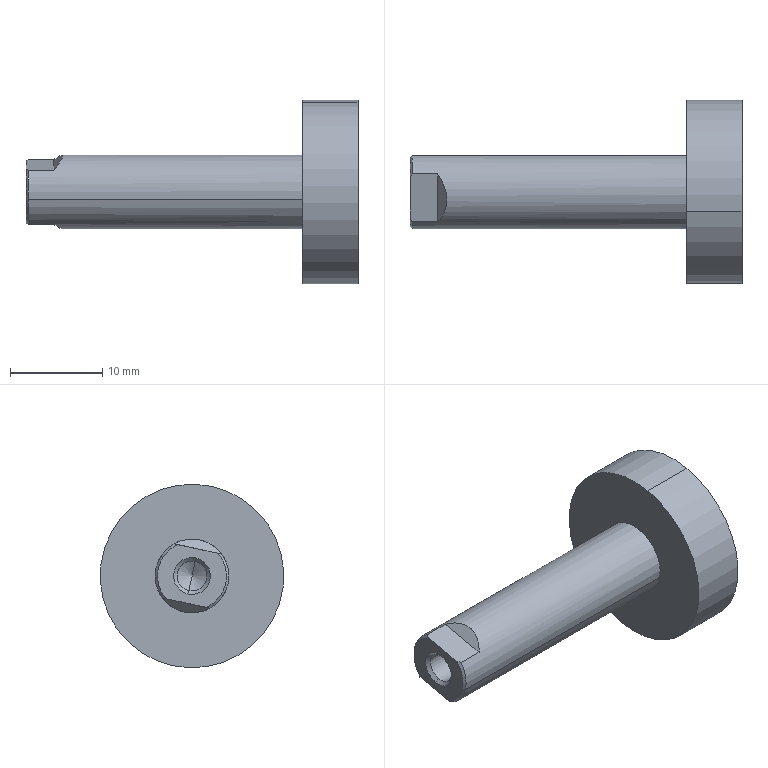Component | SolidWorks | Ultra-thinCylinderSDA2015-1_SDA2015Axis-1 | 1 solid | 19 faces | box 36 x 19.9 x 19.9 mm | volume 3266 mm3 | plane 7 | cone 6 | cylinder 6 | commonest cylinder face diameters 3.242 x2 8 x2 19.9 x2
STEP:
#1=COLOUR_RGB('',0.7922,0.8196,0.9333);
#2=FILL_AREA_STYLE_COLOUR('',#1);
#3=FILL_AREA_STYLE('',(#2));
#4=SURFACE_STYLE_FILL_AREA(#3);
#5=SURFACE_SIDE_STYLE('',(#4));
#6=SURFACE_STYLE_USAGE(.BOTH.,#5);
#7=PRESENTATION_STYLE_ASSIGNMENT((#6));
#8=CARTESIAN_POINT('',(-0.6774,1.402,-1.737));
#9=VERTEX_POINT('',#8);
#10=CARTESIAN_POINT('',(-0.6774,1.478,-1.786));
#11=VERTEX_POINT('',#10);
#12=CARTESIAN_POINT('',(-0.6774,1.464,-1.723));
#13=DIRECTION('',(1.,0.,-0.));
#14=DIRECTION('',(0.,-0.2122,0.9772));
#15=AXIS2_PLACEMENT_3D('',#12,#13,#14);
#16=CIRCLE('',#15,0.06382);
#17=EDGE_CURVE('',#9,#11,#16,.T.);
#18=ORIENTED_EDGE('',*,*,#17,.T.);
#19=CARTESIAN_POINT('',(-0.6923,1.481,-1.8));
#20=VERTEX_POINT('',#19);
#21=CARTESIAN_POINT('',(-0.6923,1.481,-1.8));
#22=DIRECTION('',(-0.7071,0.1501,-0.691));
#23=VECTOR('',#22,39.37);
#24=LINE('',#21,#23);
#25=EDGE_CURVE('',#11,#20,#24,.T.);
#26=ORIENTED_EDGE('',*,*,#25,.T.);
#27=CARTESIAN_POINT('',(-0.6923,1.447,-1.646));
#28=VERTEX_POINT('',#27);
#29=CARTESIAN_POINT('',(-0.6923,1.464,-1.723));
#30=DIRECTION('',(1.,0.,-0.));
#31=DIRECTION('',(0.,-0.2122,0.9772));
#32=AXIS2_PLACEMENT_3D('',#29,#30,#31);
#33=CIRCLE('',#32,0.07874);
#34=EDGE_CURVE('',#28,#20,#33,.T.);
#35=ORIENTED_EDGE('',*,*,#34,.F.);
#36=CARTESIAN_POINT('',(-0.6774,1.45,-1.661));
#37=VERTEX_POINT('',#36);
#38=CARTESIAN_POINT('',(-0.6923,1.447,-1.646));
#39=DIRECTION('',(-0.7071,-0.1501,0.691));
#40=VECTOR('',#39,39.37);
#41=LINE('',#38,#40);
#42=EDGE_CURVE('',#37,#28,#41,.T.);
#43=ORIENTED_EDGE('',*,*,#42,.F.);
#44=CARTESIAN_POINT('',(-0.6774,1.464,-1.723));
#45=DIRECTION('',(1.,0.,-0.));
#46=DIRECTION('',(0.,-0.2122,0.9772));
#47=AXIS2_PLACEMENT_3D('',#44,#45,#46);
#48=CIRCLE('',#47,0.06382);
#49=EDGE_CURVE('',#37,#9,#48,.T.);
#50=ORIENTED_EDGE('',*,*,#49,.T.);
#51=EDGE_LOOP('',(#18,#26,#35,#43,#50));
#52=FACE_OUTER_BOUND('',#51,.T.);
#53=CARTESIAN_POINT('',(-0.6923,1.464,-1.723));
#54=DIRECTION('',(-1.,-0.,0.));
#55=DIRECTION('',(0.,-0.2122,0.9772));
#56=AXIS2_PLACEMENT_3D('',#53,#54,#55);
#57=CONICAL_SURFACE('',#56,0.07874,0.7854);
#58=ADVANCED_FACE('',(#52),#57,.F.);
#59=ORIENTED_EDGE('',*,*,#17,.F.);
#60=CARTESIAN_POINT('',(-0.3144,1.402,-1.737));
#61=VERTEX_POINT('',#60);
#62=CARTESIAN_POINT('',(-0.6774,1.402,-1.737));
#63=DIRECTION('',(1.,-0.,-0.));
#64=VECTOR('',#63,39.37);
#65=LINE('',#62,#64);
#66=EDGE_CURVE('',#9,#61,#65,.T.);
#67=ORIENTED_EDGE('',*,*,#66,.T.);
#68=CARTESIAN_POINT('',(-0.3144,1.478,-1.786));
#69=VERTEX_POINT('',#68);
#70=CARTESIAN_POINT('',(-0.3144,1.464,-1.723));
#71=DIRECTION('',(1.,-0.,-0.));
#72=DIRECTION('',(0.,0.9772,0.2122));
#73=AXIS2_PLACEMENT_3D('',#70,#71,#72);
#74=CIRCLE('',#73,0.06382);
#75=EDGE_CURVE('',#61,#69,#74,.T.);
#76=ORIENTED_EDGE('',*,*,#75,.T.);
#77=CARTESIAN_POINT('',(-0.3144,1.526,-1.71));
#78=VERTEX_POINT('',#77);
#79=CARTESIAN_POINT('',(-0.3144,1.464,-1.723));
#80=DIRECTION('',(1.,-0.,-0.));
#81=DIRECTION('',(0.,0.9772,0.2122));
#82=AXIS2_PLACEMENT_3D('',#79,#80,#81);
#83=CIRCLE('',#82,0.06382);
#84=EDGE_CURVE('',#69,#78,#83,.T.);
#85=ORIENTED_EDGE('',*,*,#84,.T.);
#86=CARTESIAN_POINT('',(-0.6774,1.526,-1.71));
#87=VERTEX_POINT('',#86);
#88=CARTESIAN_POINT('',(-0.6774,1.526,-1.71));
#89=DIRECTION('',(1.,-0.,-0.));
#90=VECTOR('',#89,39.37);
#91=LINE('',#88,#90);
#92=EDGE_CURVE('',#87,#78,#91,.T.);
#93=ORIENTED_EDGE('',*,*,#92,.F.);
#94=CARTESIAN_POINT('',(-0.6774,1.464,-1.723));
#95=DIRECTION('',(1.,0.,-0.));
#96=DIRECTION('',(0.,-0.2122,0.9772));
#97=AXIS2_PLACEMENT_3D('',#94,#95,#96);
#98=CIRCLE('',#97,0.06382);
#99=EDGE_CURVE('',#11,#87,#98,.T.);
#100=ORIENTED_EDGE('',*,*,#99,.F.);
#101=EDGE_LOOP('',(#59,#67,#76,#85,#93,#100));
#102=FACE_OUTER_BOUND('',#101,.T.);
#103=CARTESIAN_POINT('',(-0.6774,1.464,-1.723));
#104=DIRECTION('',(1.,-0.,-0.));
#105=DIRECTION('',(0.,0.9772,0.2122));
#106=AXIS2_PLACEMENT_3D('',#103,#104,#105);
#107=CYLINDRICAL_SURFACE('',#106,0.06382);
#108=ADVANCED_FACE('',(#102),#107,.F.);
#109=CARTESIAN_POINT('',(-0.2775,1.464,-1.723));
#110=VERTEX_POINT('',#109);
#111=CARTESIAN_POINT('',(-0.3144,1.45,-1.661));
#112=VERTEX_POINT('',#111);
#113=CARTESIAN_POINT('',(-0.3144,1.45,-1.661));
#114=DIRECTION('',(-0.5,-0.1838,0.8463));
#115=VECTOR('',#114,39.37);
#116=LINE('',#113,#115);
#117=EDGE_CURVE('',#110,#112,#116,.T.);
#118=ORIENTED_EDGE('',*,*,#117,.F.);
#119=CARTESIAN_POINT('',(-0.3144,1.478,-1.786));
#120=DIRECTION('',(-0.5,0.1838,-0.8463));
#121=VECTOR('',#120,39.37);
#122=LINE('',#119,#121);
#123=EDGE_CURVE('',#110,#69,#122,.T.);
#124=ORIENTED_EDGE('',*,*,#123,.T.);
#125=ORIENTED_EDGE('',*,*,#75,.F.);
#126=CARTESIAN_POINT('',(-0.3144,1.464,-1.723));
#127=DIRECTION('',(1.,-0.,-0.));
#128=DIRECTION('',(0.,0.9772,0.2122));
#129=AXIS2_PLACEMENT_3D('',#126,#127,#128);
#130=CIRCLE('',#129,0.06382);
#131=EDGE_CURVE('',#112,#61,#130,.T.);
#132=ORIENTED_EDGE('',*,*,#131,.F.);
#133=EDGE_LOOP('',(#118,#124,#125,#132));
#134=FACE_OUTER_BOUND('',#133,.T.);
#135=CARTESIAN_POINT('',(-0.3144,1.464,-1.723));
#136=DIRECTION('',(-1.,-0.,0.));
#137=DIRECTION('',(0.,-0.2122,0.9772));
#138=AXIS2_PLACEMENT_3D('',#135,#136,#137);
#139=CONICAL_SURFACE('',#138,0.06382,1.047);
#140=ADVANCED_FACE('',(#134),#139,.F.);
#141=CARTESIAN_POINT('',(-0.6825,1.31,-1.757));
#142=VERTEX_POINT('',#141);
#143=CARTESIAN_POINT('',(-0.6825,1.337,-1.63));
#144=VERTEX_POINT('',#143);
#145=CARTESIAN_POINT('',(-0.6825,1.464,-1.723));
#146=DIRECTION('',(-1.,-0.,0.));
#147=DIRECTION('',(0.,0.2122,-0.9772));
#148=AXIS2_PLACEMENT_3D('',#145,#146,#147);
#149=CIRCLE('',#148,0.1575);
#150=EDGE_CURVE('',#142,#144,#149,.T.);
#151=ORIENTED_EDGE('',*,*,#150,.F.);
#152=CARTESIAN_POINT('',(0.4888,1.31,-1.757));
#153=VERTEX_POINT('',#152);
#154=CARTESIAN_POINT('',(0.4888,1.31,-1.757));
#155=DIRECTION('',(1.,0.,-0.));
#156=VECTOR('',#155,39.37);
#157=LINE('',#154,#156);
#158=EDGE_CURVE('',#142,#153,#157,.T.);
#159=ORIENTED_EDGE('',*,*,#158,.T.);
#160=CARTESIAN_POINT('',(0.4888,1.618,-1.69));
#161=VERTEX_POINT('',#160);
#162=CARTESIAN_POINT('',(0.4888,1.464,-1.723));
#163=DIRECTION('',(-1.,-0.,0.));
#164=DIRECTION('',(-0.,0.9772,0.2122));
#165=AXIS2_PLACEMENT_3D('',#162,#163,#164);
#166=CIRCLE('',#165,0.1575);
#167=EDGE_CURVE('',#153,#161,#166,.T.);
#168=ORIENTED_EDGE('',*,*,#167,.T.);
#169=CARTESIAN_POINT('',(-0.6825,1.618,-1.69));
#170=VERTEX_POINT('',#169);
#171=CARTESIAN_POINT('',(0.4888,1.618,-1.69));
#172=DIRECTION('',(1.,0.,-0.));
#173=VECTOR('',#172,39.37);
#174=LINE('',#171,#173);
#175=EDGE_CURVE('',#170,#161,#174,.T.);
#176=ORIENTED_EDGE('',*,*,#175,.F.);
#177=CARTESIAN_POINT('',(-0.6825,1.541,-1.586));
#178=VERTEX_POINT('',#177);
#179=CARTESIAN_POINT('',(-0.6825,1.464,-1.723));
#180=DIRECTION('',(-1.,-0.,0.));
#181=DIRECTION('',(0.,0.2122,-0.9772));
#182=AXIS2_PLACEMENT_3D('',#179,#180,#181);
#183=CIRCLE('',#182,0.1575);
#184=EDGE_CURVE('',#178,#170,#183,.T.);
#185=ORIENTED_EDGE('',*,*,#184,.F.);
#186=CARTESIAN_POINT('',(-0.5742,1.541,-1.586));
#187=VERTEX_POINT('',#186);
#188=CARTESIAN_POINT('',(-0.6333,1.541,-1.586));
#189=DIRECTION('',(-1.,-0.,0.));
#190=VECTOR('',#189,39.37);
#191=LINE('',#188,#190);
#192=EDGE_CURVE('',#187,#178,#191,.T.);
#193=ORIENTED_EDGE('',*,*,#192,.F.);
#194=CARTESIAN_POINT('',(-0.5742,1.337,-1.63));
#195=VERTEX_POINT('',#194);
#196=CARTESIAN_POINT('',(-0.5742,1.541,-1.586));
#197=CARTESIAN_POINT('',(-0.5191,1.468,-1.545));
#198=CARTESIAN_POINT('',(-0.5191,1.387,-1.563));
#199=CARTESIAN_POINT('',(-0.5742,1.337,-1.63));
#200=(BOUNDED_CURVE()B_SPLINE_CURVE(3,(#196,#197,#198,#199),.UNSPECIFIED.,.F.,.F.)B_SPLINE_CURVE_WITH_KNOTS((4,4),(5.56,7.006),.UNSPECIFIED.)CURVE()GEOMETRIC_REPRESENTATION_ITEM()RATIONAL_B_SPLINE_CURVE((1.,0.8333,0.8333,1.))REPRESENTATION_ITEM(''));
#201=EDGE_CURVE('',#187,#195,#200,.T.);
#202=ORIENTED_EDGE('',*,*,#201,.T.);
#203=CARTESIAN_POINT('',(-0.6333,1.337,-1.63));
#204=DIRECTION('',(1.,0.,-0.));
#205=VECTOR('',#204,39.37);
#206=LINE('',#203,#205);
#207=EDGE_CURVE('',#144,#195,#206,.T.);
#208=ORIENTED_EDGE('',*,*,#207,.F.);
#209=EDGE_LOOP('',(#151,#159,#168,#176,#185,#193,#202,#208));
#210=FACE_OUTER_BOUND('',#209,.T.);
#211=CARTESIAN_POINT('',(0.4888,1.464,-1.723));
#212=DIRECTION('',(1.,0.,-0.));
#213=DIRECTION('',(-0.,0.9772,0.2122));
#214=AXIS2_PLACEMENT_3D('',#211,#212,#213);
#215=CYLINDRICAL_SURFACE('',#214,0.1575);
#216=ADVANCED_FACE('',(#210),#215,.T.);
#217=CARTESIAN_POINT('',(0.4888,1.381,-1.341));
#218=VERTEX_POINT('',#217);
#219=CARTESIAN_POINT('',(0.4888,1.547,-2.106));
#220=VERTEX_POINT('',#219);
#221=CARTESIAN_POINT('',(0.4888,1.464,-1.723));
#222=DIRECTION('',(-1.,-0.,0.));
#223=DIRECTION('',(-0.,0.2122,-0.9772));
#224=AXIS2_PLACEMENT_3D('',#221,#222,#223);
#225=CIRCLE('',#224,0.3917);
#226=EDGE_CURVE('',#218,#220,#225,.T.);
#227=ORIENTED_EDGE('',*,*,#226,.F.);
#228=CARTESIAN_POINT('',(0.725,1.381,-1.341));
#229=VERTEX_POINT('',#228);
#230=CARTESIAN_POINT('',(0.725,1.381,-1.341));
#231=DIRECTION('',(1.,0.,-0.));
#232=VECTOR('',#231,39.37);
#233=LINE('',#230,#232);
#234=EDGE_CURVE('',#218,#229,#233,.T.);
#235=ORIENTED_EDGE('',*,*,#234,.T.);
#236=CARTESIAN_POINT('',(0.725,1.547,-2.106));
#237=VERTEX_POINT('',#236);
#238=CARTESIAN_POINT('',(0.725,1.464,-1.723));
#239=DIRECTION('',(-1.,-0.,0.));
#240=DIRECTION('',(0.,0.2122,-0.9772));
#241=AXIS2_PLACEMENT_3D('',#238,#239,#240);
#242=CIRCLE('',#241,0.3917);
#243=EDGE_CURVE('',#229,#237,#242,.T.);
#244=ORIENTED_EDGE('',*,*,#243,.T.);
#245=CARTESIAN_POINT('',(0.725,1.547,-2.106));
#246=DIRECTION('',(1.,0.,-0.));
#247=VECTOR('',#246,39.37);
#248=LINE('',#245,#247);
#249=EDGE_CURVE('',#220,#237,#248,.T.);
#250=ORIENTED_EDGE('',*,*,#249,.F.);
#251=EDGE_LOOP('',(#227,#235,#244,#250));
#252=FACE_OUTER_BOUND('',#251,.T.);
#253=CARTESIAN_POINT('',(0.725,1.464,-1.723));
#254=DIRECTION('',(1.,0.,-0.));
#255=DIRECTION('',(0.,0.2122,-0.9772));
#256=AXIS2_PLACEMENT_3D('',#253,#254,#255);
#257=CYLINDRICAL_SURFACE('',#256,0.3917);
#258=ADVANCED_FACE('',(#252),#257,.T.);
#259=ORIENTED_EDGE('',*,*,#25,.F.);
#260=ORIENTED_EDGE('',*,*,#99,.T.);
#261=CARTESIAN_POINT('',(-0.6774,1.464,-1.723));
#262=DIRECTION('',(1.,0.,-0.));
#263=DIRECTION('',(0.,-0.2122,0.9772));
#264=AXIS2_PLACEMENT_3D('',#261,#262,#263);
#265=CIRCLE('',#264,0.06382);
#266=EDGE_CURVE('',#87,#37,#265,.T.);
#267=ORIENTED_EDGE('',*,*,#266,.T.);
#268=ORIENTED_EDGE('',*,*,#42,.T.);
#269=CARTESIAN_POINT('',(-0.6923,1.464,-1.723));
#270=DIRECTION('',(1.,0.,-0.));
#271=DIRECTION('',(0.,-0.2122,0.9772));
#272=AXIS2_PLACEMENT_3D('',#269,#270,#271);
#273=CIRCLE('',#272,0.07874);
#274=EDGE_CURVE('',#20,#28,#273,.T.);
#275=ORIENTED_EDGE('',*,*,#274,.F.);
#276=EDGE_LOOP('',(#259,#260,#267,#268,#275));
#277=FACE_OUTER_BOUND('',#276,.T.);
#278=CARTESIAN_POINT('',(-0.6923,1.464,-1.723));
#279=DIRECTION('',(-1.,-0.,0.));
#280=DIRECTION('',(0.,-0.2122,0.9772));
#281=AXIS2_PLACEMENT_3D('',#278,#279,#280);
#282=CONICAL_SURFACE('',#281,0.07874,0.7854);
#283=ADVANCED_FACE('',(#277),#282,.F.);
#284=ORIENTED_EDGE('',*,*,#66,.F.);
#285=ORIENTED_EDGE('',*,*,#49,.F.);
#286=ORIENTED_EDGE('',*,*,#266,.F.);
#287=ORIENTED_EDGE('',*,*,#92,.T.);
#288=CARTESIAN_POINT('',(-0.3144,1.464,-1.723));
#289=DIRECTION('',(1.,-0.,-0.));
#290=DIRECTION('',(0.,0.9772,0.2122));
#291=AXIS2_PLACEMENT_3D('',#288,#289,#290);
#292=CIRCLE('',#291,0.06382);
#293=EDGE_CURVE('',#78,#112,#292,.T.);
#294=ORIENTED_EDGE('',*,*,#293,.T.);
#295=ORIENTED_EDGE('',*,*,#131,.T.);
#296=EDGE_LOOP('',(#284,#285,#286,#287,#294,#295));
#297=FACE_OUTER_BOUND('',#296,.T.);
#298=CARTESIAN_POINT('',(-0.6774,1.464,-1.723));
#299=DIRECTION('',(1.,-0.,-0.));
#300=DIRECTION('',(0.,0.9772,0.2122));
#301=AXIS2_PLACEMENT_3D('',#298,#299,#300);
#302=CYLINDRICAL_SURFACE('',#301,0.06382);
#303=ADVANCED_FACE('',(#297),#302,.F.);
#304=ORIENTED_EDGE('',*,*,#123,.F.);
#305=ORIENTED_EDGE('',*,*,#117,.T.);
#306=ORIENTED_EDGE('',*,*,#293,.F.);
#307=ORIENTED_EDGE('',*,*,#84,.F.);
#308=EDGE_LOOP('',(#304,#305,#306,#307));
#309=FACE_OUTER_BOUND('',#308,.T.);
#310=CARTESIAN_POINT('',(-0.3144,1.464,-1.723));
#311=DIRECTION('',(-1.,-0.,0.));
#312=DIRECTION('',(0.,-0.2122,0.9772));
#313=AXIS2_PLACEMENT_3D('',#310,#311,#312);
#314=CONICAL_SURFACE('',#313,0.06382,1.047);
#315=ADVANCED_FACE('',(#309),#314,.F.);
#316=ORIENTED_EDGE('',*,*,#34,.T.);
#317=ORIENTED_EDGE('',*,*,#274,.T.);
#318=EDGE_LOOP('',(#316,#317));
#319=FACE_BOUND('',#318,.T.);
#320=CARTESIAN_POINT('',(-0.6923,1.402,-1.858));
#321=VERTEX_POINT('',#320);
#322=CARTESIAN_POINT('',(-0.6923,1.352,-1.627));
#323=VERTEX_POINT('',#322);
#324=CARTESIAN_POINT('',(-0.6923,1.464,-1.723));
#325=DIRECTION('',(-1.,-0.,0.));
#326=DIRECTION('',(0.,0.2122,-0.9772));
#327=AXIS2_PLACEMENT_3D('',#324,#325,#326);
#328=CIRCLE('',#327,0.1476);
#329=EDGE_CURVE('',#321,#323,#328,.T.);
#330=ORIENTED_EDGE('',*,*,#329,.T.);
#331=CARTESIAN_POINT('',(-0.6923,1.525,-1.589));
#332=VERTEX_POINT('',#331);
#333=CARTESIAN_POINT('',(-0.6923,1.293,-1.64));
#334=DIRECTION('',(0.,0.9772,0.2122));
#335=VECTOR('',#334,39.37);
#336=LINE('',#333,#335);
#337=EDGE_CURVE('',#323,#332,#336,.T.);
#338=ORIENTED_EDGE('',*,*,#337,.T.);
#339=CARTESIAN_POINT('',(-0.6923,1.576,-1.82));
#340=VERTEX_POINT('',#339);
#341=CARTESIAN_POINT('',(-0.6923,1.464,-1.723));
#342=DIRECTION('',(-1.,-0.,0.));
#343=DIRECTION('',(0.,0.2122,-0.9772));
#344=AXIS2_PLACEMENT_3D('',#341,#342,#343);
#345=CIRCLE('',#344,0.1476);
#346=EDGE_CURVE('',#332,#340,#345,.T.);
#347=ORIENTED_EDGE('',*,*,#346,.T.);
#348=CARTESIAN_POINT('',(-0.6923,1.343,-1.871));
#349=DIRECTION('',(-0.,-0.9772,-0.2122));
#350=VECTOR('',#349,39.37);
#351=LINE('',#348,#350);
#352=EDGE_CURVE('',#340,#321,#351,.T.);
#353=ORIENTED_EDGE('',*,*,#352,.T.);
#354=EDGE_LOOP('',(#330,#338,#347,#353));
#355=FACE_OUTER_BOUND('',#354,.T.);
#356=CARTESIAN_POINT('',(-0.6923,1.343,-1.871));
#357=DIRECTION('',(-1.,-0.,0.));
#358=DIRECTION('',(0.,-0.2122,0.9772));
#359=AXIS2_PLACEMENT_3D('',#356,#357,#358);
#360=PLANE('',#359);
#361=ADVANCED_FACE('',(#319,#355),#360,.T.);
#362=CARTESIAN_POINT('',(-0.6825,1.541,-1.586));
#363=CARTESIAN_POINT('',(-0.686,1.535,-1.587));
#364=CARTESIAN_POINT('',(-0.6893,1.53,-1.588));
#365=CARTESIAN_POINT('',(-0.6923,1.525,-1.589));
#366=B_SPLINE_CURVE_WITH_KNOTS('',3,(#362,#363,#364,#365),.UNSPECIFIED.,.F.,.F.,(4,4),(0.007414,0.007883),.UNSPECIFIED.);
#367=EDGE_CURVE('',#178,#332,#366,.T.);
#368=ORIENTED_EDGE('',*,*,#367,.T.);
#369=ORIENTED_EDGE('',*,*,#337,.F.);
#370=CARTESIAN_POINT('',(-0.6923,1.352,-1.627));
#371=CARTESIAN_POINT('',(-0.6893,1.347,-1.628));
#372=CARTESIAN_POINT('',(-0.686,1.342,-1.629));
#373=CARTESIAN_POINT('',(-0.6825,1.337,-1.63));
#374=B_SPLINE_CURVE_WITH_KNOTS('',3,(#370,#371,#372,#373),.UNSPECIFIED.,.F.,.F.,(4,4),(0.01265,0.01312),.UNSPECIFIED.);
#375=EDGE_CURVE('',#323,#144,#374,.T.);
#376=ORIENTED_EDGE('',*,*,#375,.T.);
#377=ORIENTED_EDGE('',*,*,#207,.T.);
#378=CARTESIAN_POINT('',(-0.5742,1.337,-1.63));
#379=DIRECTION('',(0.,0.9772,0.2122));
#380=VECTOR('',#379,39.37);
#381=LINE('',#378,#380);
#382=EDGE_CURVE('',#195,#187,#381,.T.);
#383=ORIENTED_EDGE('',*,*,#382,.T.);
#384=ORIENTED_EDGE('',*,*,#192,.T.);
#385=EDGE_LOOP('',(#368,#369,#376,#377,#383,#384));
#386=FACE_OUTER_BOUND('',#385,.T.);
#387=CARTESIAN_POINT('',(-0.6923,1.337,-1.63));
#388=DIRECTION('',(0.,-0.2122,0.9772));
#389=DIRECTION('',(1.,0.,-0.));
#390=AXIS2_PLACEMENT_3D('',#387,#388,#389);
#391=PLANE('',#390);
#392=ADVANCED_FACE('',(#386),#391,.T.);
#393=CARTESIAN_POINT('',(-0.6825,1.387,-1.861));
#394=VERTEX_POINT('',#393);
#395=CARTESIAN_POINT('',(-0.6923,1.402,-1.858));
#396=CARTESIAN_POINT('',(-0.6893,1.398,-1.859));
#397=CARTESIAN_POINT('',(-0.686,1.392,-1.86));
#398=CARTESIAN_POINT('',(-0.6825,1.387,-1.861));
#399=B_SPLINE_CURVE_WITH_KNOTS('',3,(#395,#396,#397,#398),.UNSPECIFIED.,.F.,.F.,(4,4),(-0.007883,-0.007414),.UNSPECIFIED.);
#400=EDGE_CURVE('',#321,#394,#399,.T.);
#401=ORIENTED_EDGE('',*,*,#400,.T.);
#402=CARTESIAN_POINT('',(-0.6825,1.464,-1.723));
#403=DIRECTION('',(-1.,-0.,0.));
#404=DIRECTION('',(0.,0.2122,-0.9772));
#405=AXIS2_PLACEMENT_3D('',#402,#403,#404);
#406=CIRCLE('',#405,0.1575);
#407=EDGE_CURVE('',#394,#142,#406,.T.);
#408=ORIENTED_EDGE('',*,*,#407,.T.);
#409=ORIENTED_EDGE('',*,*,#150,.T.);
#410=ORIENTED_EDGE('',*,*,#375,.F.);
#411=ORIENTED_EDGE('',*,*,#329,.F.);
#412=EDGE_LOOP('',(#401,#408,#409,#410,#411));
#413=FACE_OUTER_BOUND('',#412,.T.);
#414=CARTESIAN_POINT('',(-0.6923,1.464,-1.723));
#415=DIRECTION('',(1.,0.,-0.));
#416=DIRECTION('',(0.,0.2122,-0.9772));
#417=AXIS2_PLACEMENT_3D('',#414,#415,#416);
#418=CONICAL_SURFACE('',#417,0.1476,0.7854);
#419=ADVANCED_FACE('',(#413),#418,.T.);
#420=ORIENTED_EDGE('',*,*,#400,.F.);
#421=ORIENTED_EDGE('',*,*,#352,.F.);
#422=CARTESIAN_POINT('',(-0.6825,1.591,-1.817));
#423=VERTEX_POINT('',#422);
#424=CARTESIAN_POINT('',(-0.6923,1.576,-1.82));
#425=CARTESIAN_POINT('',(-0.6893,1.581,-1.819));
#426=CARTESIAN_POINT('',(-0.686,1.586,-1.818));
#427=CARTESIAN_POINT('',(-0.6825,1.591,-1.817));
#428=B_SPLINE_CURVE_WITH_KNOTS('',3,(#424,#425,#426,#427),.UNSPECIFIED.,.F.,.F.,(4,4),(0.01265,0.01312),.UNSPECIFIED.);
#429=EDGE_CURVE('',#340,#423,#428,.T.);
#430=ORIENTED_EDGE('',*,*,#429,.T.);
#431=CARTESIAN_POINT('',(-0.5742,1.591,-1.817));
#432=VERTEX_POINT('',#431);
#433=CARTESIAN_POINT('',(-0.6333,1.591,-1.817));
#434=DIRECTION('',(1.,0.,-0.));
#435=VECTOR('',#434,39.37);
#436=LINE('',#433,#435);
#437=EDGE_CURVE('',#423,#432,#436,.T.);
#438=ORIENTED_EDGE('',*,*,#437,.T.);
#439=CARTESIAN_POINT('',(-0.5742,1.387,-1.861));
#440=VERTEX_POINT('',#439);
#441=CARTESIAN_POINT('',(-0.5742,1.387,-1.861));
#442=DIRECTION('',(-0.,-0.9772,-0.2122));
#443=VECTOR('',#442,39.37);
#444=LINE('',#441,#443);
#445=EDGE_CURVE('',#432,#440,#444,.T.);
#446=ORIENTED_EDGE('',*,*,#445,.T.);
#447=CARTESIAN_POINT('',(-0.6333,1.387,-1.861));
#448=DIRECTION('',(-1.,-0.,0.));
#449=VECTOR('',#448,39.37);
#450=LINE('',#447,#449);
#451=EDGE_CURVE('',#440,#394,#450,.T.);
#452=ORIENTED_EDGE('',*,*,#451,.T.);
#453=EDGE_LOOP('',(#420,#421,#430,#438,#446,#452));
#454=FACE_OUTER_BOUND('',#453,.T.);
#455=CARTESIAN_POINT('',(-0.5742,1.387,-1.861));
#456=DIRECTION('',(-0.,0.2122,-0.9772));
#457=DIRECTION('',(-1.,-0.,0.));
#458=AXIS2_PLACEMENT_3D('',#455,#456,#457);
#459=PLANE('',#458);
#460=ADVANCED_FACE('',(#454),#459,.T.);
#461=ORIENTED_EDGE('',*,*,#367,.F.);
#462=ORIENTED_EDGE('',*,*,#184,.T.);
#463=CARTESIAN_POINT('',(-0.6825,1.464,-1.723));
#464=DIRECTION('',(-1.,-0.,0.));
#465=DIRECTION('',(0.,0.2122,-0.9772));
#466=AXIS2_PLACEMENT_3D('',#463,#464,#465);
#467=CIRCLE('',#466,0.1575);
#468=EDGE_CURVE('',#170,#423,#467,.T.);
#469=ORIENTED_EDGE('',*,*,#468,.T.);
#470=ORIENTED_EDGE('',*,*,#429,.F.);
#471=ORIENTED_EDGE('',*,*,#346,.F.);
#472=EDGE_LOOP('',(#461,#462,#469,#470,#471));
#473=FACE_OUTER_BOUND('',#472,.T.);
#474=CARTESIAN_POINT('',(-0.6923,1.464,-1.723));
#475=DIRECTION('',(1.,0.,-0.));
#476=DIRECTION('',(0.,0.2122,-0.9772));
#477=AXIS2_PLACEMENT_3D('',#474,#475,#476);
#478=CONICAL_SURFACE('',#477,0.1476,0.7854);
#479=ADVANCED_FACE('',(#473),#478,.T.);
#480=ORIENTED_EDGE('',*,*,#158,.F.);
#481=ORIENTED_EDGE('',*,*,#407,.F.);
#482=ORIENTED_EDGE('',*,*,#451,.F.);
#483=CARTESIAN_POINT('',(-0.5742,1.387,-1.861));
#484=CARTESIAN_POINT('',(-0.5191,1.46,-1.902));
#485=CARTESIAN_POINT('',(-0.5191,1.541,-1.884));
#486=CARTESIAN_POINT('',(-0.5742,1.591,-1.817));
#487=(BOUNDED_CURVE()B_SPLINE_CURVE(3,(#483,#484,#485,#486),.UNSPECIFIED.,.F.,.F.)B_SPLINE_CURVE_WITH_KNOTS((4,4),(5.56,7.006),.UNSPECIFIED.)CURVE()GEOMETRIC_REPRESENTATION_ITEM()RATIONAL_B_SPLINE_CURVE((1.,0.8333,0.8333,1.))REPRESENTATION_ITEM(''));
#488=EDGE_CURVE('',#440,#432,#487,.T.);
#489=ORIENTED_EDGE('',*,*,#488,.T.);
#490=ORIENTED_EDGE('',*,*,#437,.F.);
#491=ORIENTED_EDGE('',*,*,#468,.F.);
#492=ORIENTED_EDGE('',*,*,#175,.T.);
#493=CARTESIAN_POINT('',(0.4888,1.464,-1.723));
#494=DIRECTION('',(-1.,-0.,0.));
#495=DIRECTION('',(-0.,0.9772,0.2122));
#496=AXIS2_PLACEMENT_3D('',#493,#494,#495);
#497=CIRCLE('',#496,0.1575);
#498=EDGE_CURVE('',#161,#153,#497,.T.);
#499=ORIENTED_EDGE('',*,*,#498,.T.);
#500=EDGE_LOOP('',(#480,#481,#482,#489,#490,#491,#492,#499));
#501=FACE_OUTER_BOUND('',#500,.T.);
#502=CARTESIAN_POINT('',(0.4888,1.464,-1.723));
#503=DIRECTION('',(1.,0.,-0.));
#504=DIRECTION('',(-0.,0.9772,0.2122));
#505=AXIS2_PLACEMENT_3D('',#502,#503,#504);
#506=CYLINDRICAL_SURFACE('',#505,0.1575);
#507=ADVANCED_FACE('',(#501),#506,.T.);
#508=ORIENTED_EDGE('',*,*,#201,.F.);
#509=ORIENTED_EDGE('',*,*,#382,.F.);
#510=EDGE_LOOP('',(#508,#509));
#511=FACE_OUTER_BOUND('',#510,.T.);
#512=CARTESIAN_POINT('',(-0.5742,1.336,-1.63));
#513=DIRECTION('',(-0.7071,-0.1501,0.691));
#514=DIRECTION('',(0.7071,-0.1501,0.691));
#515=AXIS2_PLACEMENT_3D('',#512,#513,#514);
#516=PLANE('',#515);
#517=ADVANCED_FACE('',(#511),#516,.T.);
#518=ORIENTED_EDGE('',*,*,#488,.F.);
#519=ORIENTED_EDGE('',*,*,#445,.F.);
#520=EDGE_LOOP('',(#518,#519));
#521=FACE_OUTER_BOUND('',#520,.T.);
#522=CARTESIAN_POINT('',(-0.5346,1.394,-1.9));
#523=DIRECTION('',(-0.7071,0.1501,-0.691));
#524=DIRECTION('',(-0.7071,-0.1501,0.691));
#525=AXIS2_PLACEMENT_3D('',#522,#523,#524);
#526=PLANE('',#525);
#527=ADVANCED_FACE('',(#521),#526,.T.);
#528=ORIENTED_EDGE('',*,*,#498,.F.);
#529=ORIENTED_EDGE('',*,*,#167,.F.);
#530=EDGE_LOOP('',(#528,#529));
#531=FACE_BOUND('',#530,.T.);
#532=CARTESIAN_POINT('',(0.4888,1.464,-1.723));
#533=DIRECTION('',(-1.,-0.,0.));
#534=DIRECTION('',(-0.,0.2122,-0.9772));
#535=AXIS2_PLACEMENT_3D('',#532,#533,#534);
#536=CIRCLE('',#535,0.3917);
#537=EDGE_CURVE('',#220,#218,#536,.T.);
#538=ORIENTED_EDGE('',*,*,#537,.T.);
#539=ORIENTED_EDGE('',*,*,#226,.T.);
#540=EDGE_LOOP('',(#538,#539));
#541=FACE_OUTER_BOUND('',#540,.T.);
#542=CARTESIAN_POINT('',(0.4888,1.161,-2.195));
#543=DIRECTION('',(-1.,-0.,0.));
#544=DIRECTION('',(0.,-0.2122,0.9772));
#545=AXIS2_PLACEMENT_3D('',#542,#543,#544);
#546=PLANE('',#545);
#547=ADVANCED_FACE('',(#531,#541),#546,.T.);
#548=ORIENTED_EDGE('',*,*,#234,.F.);
#549=ORIENTED_EDGE('',*,*,#537,.F.);
#550=ORIENTED_EDGE('',*,*,#249,.T.);
#551=CARTESIAN_POINT('',(0.725,1.464,-1.723));
#552=DIRECTION('',(-1.,-0.,0.));
#553=DIRECTION('',(0.,0.2122,-0.9772));
#554=AXIS2_PLACEMENT_3D('',#551,#552,#553);
#555=CIRCLE('',#554,0.3917);
#556=EDGE_CURVE('',#237,#229,#555,.T.);
#557=ORIENTED_EDGE('',*,*,#556,.T.);
#558=EDGE_LOOP('',(#548,#549,#550,#557));
#559=FACE_OUTER_BOUND('',#558,.T.);
#560=CARTESIAN_POINT('',(0.725,1.464,-1.723));
#561=DIRECTION('',(1.,0.,-0.));
#562=DIRECTION('',(0.,0.2122,-0.9772));
#563=AXIS2_PLACEMENT_3D('',#560,#561,#562);
#564=CYLINDRICAL_SURFACE('',#563,0.3917);
#565=ADVANCED_FACE('',(#559),#564,.T.);
#566=ORIENTED_EDGE('',*,*,#556,.F.);
#567=ORIENTED_EDGE('',*,*,#243,.F.);
#568=EDGE_LOOP('',(#566,#567));
#569=FACE_OUTER_BOUND('',#568,.T.);
#570=CARTESIAN_POINT('',(0.725,0.9925,-1.42));
#571=DIRECTION('',(1.,0.,-0.));
#572=DIRECTION('',(-0.,0.2122,-0.9772));
#573=AXIS2_PLACEMENT_3D('',#570,#571,#572);
#574=PLANE('',#573);
#575=ADVANCED_FACE('',(#569),#574,.T.);
#576=CLOSED_SHELL('',(#58,#108,#140,#216,#258,#283,#303,#315,#361,#392,#419,#460,#479,#507,#517,#527,#547,#565,#575));
#577=MANIFOLD_SOLID_BREP('',#576);
#578=STYLED_ITEM('',(#7),#577);
#579=(LENGTH_UNIT()NAMED_UNIT(*)SI_UNIT($,.METRE.));
#580=LENGTH_MEASURE_WITH_UNIT(LENGTH_MEASURE(0.0254),#579);
#581=DIMENSIONAL_EXPONENTS(1.,0.,0.,0.,0.,0.,0.);
#582=(CONVERSION_BASED_UNIT('',#580)LENGTH_UNIT()NAMED_UNIT(#581));
#583=UNCERTAINTY_MEASURE_WITH_UNIT(LENGTH_MEASURE(0.00001),#582,'','');
#584=(NAMED_UNIT(*)PLANE_ANGLE_UNIT()SI_UNIT($,.RADIAN.));
#585=(NAMED_UNIT(*)SI_UNIT($,.STERADIAN.)SOLID_ANGLE_UNIT());
#586=(GEOMETRIC_REPRESENTATION_CONTEXT(3)GLOBAL_UNCERTAINTY_ASSIGNED_CONTEXT((#583))GLOBAL_UNIT_ASSIGNED_CONTEXT((#582,#584,#585))REPRESENTATION_CONTEXT('',''));
#587=MECHANICAL_DESIGN_GEOMETRIC_PRESENTATION_REPRESENTATION('',(#578),#586);
#588=PRESENTATION_LAYER_ASSIGNMENT('','',(#578));
#589=CARTESIAN_POINT('',(0.,0.,0.));
#590=DIRECTION('',(0.,0.,1.));
#591=DIRECTION('',(1.,0.,0.));
#592=AXIS2_PLACEMENT_3D('',#589,#590,#591);
#593=(LENGTH_UNIT()NAMED_UNIT(*)SI_UNIT($,.METRE.));
#594=LENGTH_MEASURE_WITH_UNIT(LENGTH_MEASURE(0.0254),#593);
#595=DIMENSIONAL_EXPONENTS(1.,0.,0.,0.,0.,0.,0.);
#596=(CONVERSION_BASED_UNIT('',#594)LENGTH_UNIT()NAMED_UNIT(#595));
#597=UNCERTAINTY_MEASURE_WITH_UNIT(LENGTH_MEASURE(0.00001),#596,'','');
#598=(NAMED_UNIT(*)PLANE_ANGLE_UNIT()SI_UNIT($,.RADIAN.));
#599=(NAMED_UNIT(*)SI_UNIT($,.STERADIAN.)SOLID_ANGLE_UNIT());
#600=(GEOMETRIC_REPRESENTATION_CONTEXT(3)GLOBAL_UNCERTAINTY_ASSIGNED_CONTEXT((#597))GLOBAL_UNIT_ASSIGNED_CONTEXT((#596,#598,#599))REPRESENTATION_CONTEXT('',''));
#601=ADVANCED_BREP_SHAPE_REPRESENTATION('',(#577,#592),#600);